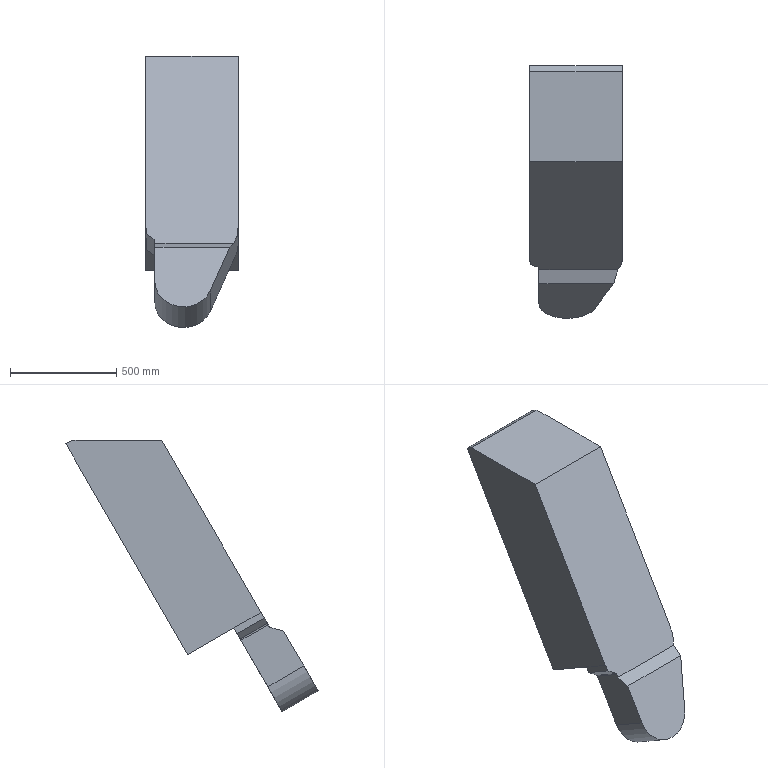Component | NX | SIM15_B1_ACHSE_DECKEL | 1 solid | 20 faces | volume 208311568 mm3 | plane 16 | cylinder 4 | commonest cylinder face diameters 20 x2 270 x1 200 x1